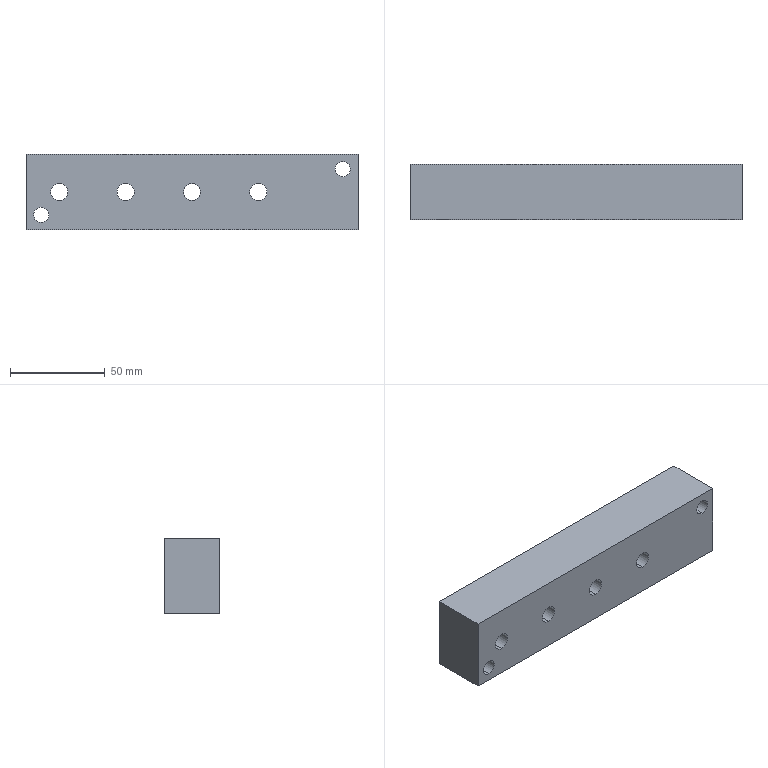Component | SolidWorks | Box151BackingPlateDiamondPin-1 | 1 solid | 33 faces | box 175 x 29 x 40 mm | volume 187063 mm3 | cylinder 22 | plane 11 | commonest cylinder face diameters 15 x8 9 x8 8 x4 10 x2
build123d program:
from build123d import *

# Parameters (mm, degrees)
SKETCH1_W                                       = 175
SKETCH1_H                                       = 40
BOSS_EXTRUDE1_DEPTH                             = 29
SKETCH2_R                                       = 5
CUT_EXTRUDE1_DEPTH                              = 20
M8_HEX_SOCKET_HEAD_CAP_SCREW_CBORE1_D           = 9
M8_HEX_SOCKET_HEAD_CAP_SCREW_CBORE1_CBORE_D     = 15
M8_HEX_SOCKET_HEAD_CAP_SCREW_CBORE1_CBORE_DEPTH = 9
SKETCH6_R                                       = 4
CUT_EXTRUDE2_DEPTH                              = 50


with BuildPart() as part:
    # Sketch1 → Boss-Extrude1 (new body)
    with BuildSketch(Plane(origin=(0, 0, 0), x_dir=(1, 0, 0), z_dir=(0, 1, 0))):
        Rectangle(SKETCH1_W, SKETCH1_H)
    extrude(amount=BOSS_EXTRUDE1_DEPTH)

    # Sketch2 → Cut-Extrude1 (cut)
    with BuildSketch(Plane(origin=(0, 29, 0), x_dir=(1, 0, 0), z_dir=(0, 1, 0))):
        with Locations(Location((-67, 2, 0), (0, 0, 270))):
            Circle(SKETCH2_R)
    extrude(amount=-CUT_EXTRUDE1_DEPTH, mode=Mode.SUBTRACT)

    # M8 Hex Socket Head Cap Screw CBORE1 (through all)
    with Locations(Plane(origin=(0, 29, 0), x_dir=(1, 0, 0), z_dir=(0, 1, 0))):
        with Locations((-35, 0), (0, 0), (35, 0), (70, 0)):
            CounterBoreHole(M8_HEX_SOCKET_HEAD_CAP_SCREW_CBORE1_D / 2, M8_HEX_SOCKET_HEAD_CAP_SCREW_CBORE1_CBORE_D / 2, M8_HEX_SOCKET_HEAD_CAP_SCREW_CBORE1_CBORE_DEPTH)

    # Sketch6 → Cut-Extrude2 (cut)
    with BuildSketch(Plane(origin=(0, 29, 0), x_dir=(1, 0, 0), z_dir=(0, 1, 0))):
        with Locations(Location((-79.5, 12, 0), (0, 0, 270))):
            Circle(SKETCH6_R)
        with Locations(Location((79.5, -12, 0), (0, 0, 270))):
            Circle(SKETCH6_R)
    extrude(amount=-CUT_EXTRUDE2_DEPTH, mode=Mode.SUBTRACT)


solid = part.part

# Placed as in the assembly
solid = solid.moved(Location((-3.619, 64.047, 50), (-180, 0, 180)))
STEP:
#1=CARTESIAN_POINT('',(2.987,2.522,2.283));
#2=VERTEX_POINT('',#1);
#3=CARTESIAN_POINT('',(2.987,2.522,2.598));
#4=VERTEX_POINT('',#3);
#5=CARTESIAN_POINT('',(2.987,2.522,2.441));
#6=DIRECTION('',(0.,-1.,0.));
#7=DIRECTION('',(0.,0.,1.));
#8=AXIS2_PLACEMENT_3D('',#5,#6,#7);
#9=CIRCLE('',#8,0.1575);
#10=EDGE_CURVE('',#2,#4,#9,.T.);
#11=ORIENTED_EDGE('',*,*,#10,.T.);
#12=CARTESIAN_POINT('',(2.987,3.663,2.598));
#13=VERTEX_POINT('',#12);
#14=CARTESIAN_POINT('',(2.987,1.695,2.598));
#15=DIRECTION('',(0.,1.,0.));
#16=VECTOR('',#15,39.37);
#17=LINE('',#14,#16);
#18=EDGE_CURVE('',#4,#13,#17,.T.);
#19=ORIENTED_EDGE('',*,*,#18,.T.);
#20=CARTESIAN_POINT('',(2.987,3.663,2.283));
#21=VERTEX_POINT('',#20);
#22=CARTESIAN_POINT('',(2.987,3.663,2.441));
#23=DIRECTION('',(0.,1.,0.));
#24=DIRECTION('',(0.,0.,-1.));
#25=AXIS2_PLACEMENT_3D('',#22,#23,#24);
#26=CIRCLE('',#25,0.1575);
#27=EDGE_CURVE('',#13,#21,#26,.T.);
#28=ORIENTED_EDGE('',*,*,#27,.T.);
#29=CARTESIAN_POINT('',(2.987,1.695,2.283));
#30=DIRECTION('',(0.,1.,0.));
#31=VECTOR('',#30,39.37);
#32=LINE('',#29,#31);
#33=EDGE_CURVE('',#2,#21,#32,.T.);
#34=ORIENTED_EDGE('',*,*,#33,.F.);
#35=EDGE_LOOP('',(#11,#19,#28,#34));
#36=FACE_OUTER_BOUND('',#35,.T.);
#37=CARTESIAN_POINT('',(2.987,1.695,2.441));
#38=DIRECTION('',(0.,1.,0.));
#39=DIRECTION('',(0.,0.,-1.));
#40=AXIS2_PLACEMENT_3D('',#37,#38,#39);
#41=CYLINDRICAL_SURFACE('',#40,0.1575);
#42=ADVANCED_FACE('',(#36),#41,.F.);
#43=CARTESIAN_POINT('',(-3.272,2.522,1.339));
#44=VERTEX_POINT('',#43);
#45=CARTESIAN_POINT('',(-3.272,2.522,1.654));
#46=VERTEX_POINT('',#45);
#47=CARTESIAN_POINT('',(-3.272,2.522,1.496));
#48=DIRECTION('',(0.,-1.,0.));
#49=DIRECTION('',(0.,0.,1.));
#50=AXIS2_PLACEMENT_3D('',#47,#48,#49);
#51=CIRCLE('',#50,0.1575);
#52=EDGE_CURVE('',#44,#46,#51,.T.);
#53=ORIENTED_EDGE('',*,*,#52,.T.);
#54=CARTESIAN_POINT('',(-3.272,3.663,1.654));
#55=VERTEX_POINT('',#54);
#56=CARTESIAN_POINT('',(-3.272,1.695,1.654));
#57=DIRECTION('',(0.,1.,0.));
#58=VECTOR('',#57,39.37);
#59=LINE('',#56,#58);
#60=EDGE_CURVE('',#46,#55,#59,.T.);
#61=ORIENTED_EDGE('',*,*,#60,.T.);
#62=CARTESIAN_POINT('',(-3.272,3.663,1.339));
#63=VERTEX_POINT('',#62);
#64=CARTESIAN_POINT('',(-3.272,3.663,1.496));
#65=DIRECTION('',(0.,1.,0.));
#66=DIRECTION('',(0.,0.,-1.));
#67=AXIS2_PLACEMENT_3D('',#64,#65,#66);
#68=CIRCLE('',#67,0.1575);
#69=EDGE_CURVE('',#55,#63,#68,.T.);
#70=ORIENTED_EDGE('',*,*,#69,.T.);
#71=CARTESIAN_POINT('',(-3.272,1.695,1.339));
#72=DIRECTION('',(0.,1.,0.));
#73=VECTOR('',#72,39.37);
#74=LINE('',#71,#73);
#75=EDGE_CURVE('',#44,#63,#74,.T.);
#76=ORIENTED_EDGE('',*,*,#75,.F.);
#77=EDGE_LOOP('',(#53,#61,#70,#76));
#78=FACE_OUTER_BOUND('',#77,.T.);
#79=CARTESIAN_POINT('',(-3.272,1.695,1.496));
#80=DIRECTION('',(0.,1.,0.));
#81=DIRECTION('',(0.,0.,-1.));
#82=AXIS2_PLACEMENT_3D('',#79,#80,#81);
#83=CYLINDRICAL_SURFACE('',#82,0.1575);
#84=ADVANCED_FACE('',(#78),#83,.F.);
#85=CARTESIAN_POINT('',(1.235,3.309,2.264));
#86=VERTEX_POINT('',#85);
#87=CARTESIAN_POINT('',(1.235,3.309,1.673));
#88=VERTEX_POINT('',#87);
#89=CARTESIAN_POINT('',(1.235,3.309,1.969));
#90=DIRECTION('',(0.,1.,0.));
#91=DIRECTION('',(0.,0.,-1.));
#92=AXIS2_PLACEMENT_3D('',#89,#90,#91);
#93=CIRCLE('',#92,0.2953);
#94=EDGE_CURVE('',#86,#88,#93,.T.);
#95=ORIENTED_EDGE('',*,*,#94,.F.);
#96=CARTESIAN_POINT('',(1.235,3.663,2.264));
#97=VERTEX_POINT('',#96);
#98=CARTESIAN_POINT('',(1.235,3.663,2.264));
#99=DIRECTION('',(0.,1.,0.));
#100=VECTOR('',#99,39.37);
#101=LINE('',#98,#100);
#102=EDGE_CURVE('',#86,#97,#101,.T.);
#103=ORIENTED_EDGE('',*,*,#102,.T.);
#104=CARTESIAN_POINT('',(1.235,3.663,1.673));
#105=VERTEX_POINT('',#104);
#106=CARTESIAN_POINT('',(1.235,3.663,1.969));
#107=DIRECTION('',(0.,1.,0.));
#108=DIRECTION('',(0.,0.,-1.));
#109=AXIS2_PLACEMENT_3D('',#106,#107,#108);
#110=CIRCLE('',#109,0.2953);
#111=EDGE_CURVE('',#97,#105,#110,.T.);
#112=ORIENTED_EDGE('',*,*,#111,.T.);
#113=CARTESIAN_POINT('',(1.235,3.663,1.673));
#114=DIRECTION('',(0.,1.,0.));
#115=VECTOR('',#114,39.37);
#116=LINE('',#113,#115);
#117=EDGE_CURVE('',#88,#105,#116,.T.);
#118=ORIENTED_EDGE('',*,*,#117,.F.);
#119=EDGE_LOOP('',(#95,#103,#112,#118));
#120=FACE_OUTER_BOUND('',#119,.T.);
#121=CARTESIAN_POINT('',(1.235,3.663,1.969));
#122=DIRECTION('',(0.,1.,0.));
#123=DIRECTION('',(0.,0.,-1.));
#124=AXIS2_PLACEMENT_3D('',#121,#122,#123);
#125=CYLINDRICAL_SURFACE('',#124,0.2953);
#126=ADVANCED_FACE('',(#120),#125,.F.);
#127=CARTESIAN_POINT('',(1.235,2.522,1.791));
#128=VERTEX_POINT('',#127);
#129=CARTESIAN_POINT('',(1.235,2.522,2.146));
#130=VERTEX_POINT('',#129);
#131=CARTESIAN_POINT('',(1.235,2.522,1.969));
#132=DIRECTION('',(0.,-1.,0.));
#133=DIRECTION('',(0.,0.,1.));
#134=AXIS2_PLACEMENT_3D('',#131,#132,#133);
#135=CIRCLE('',#134,0.1772);
#136=EDGE_CURVE('',#128,#130,#135,.T.);
#137=ORIENTED_EDGE('',*,*,#136,.T.);
#138=CARTESIAN_POINT('',(1.235,3.309,2.146));
#139=VERTEX_POINT('',#138);
#140=CARTESIAN_POINT('',(1.235,3.663,2.146));
#141=DIRECTION('',(0.,1.,0.));
#142=VECTOR('',#141,39.37);
#143=LINE('',#140,#142);
#144=EDGE_CURVE('',#130,#139,#143,.T.);
#145=ORIENTED_EDGE('',*,*,#144,.T.);
#146=CARTESIAN_POINT('',(1.235,3.309,1.791));
#147=VERTEX_POINT('',#146);
#148=CARTESIAN_POINT('',(1.235,3.309,1.969));
#149=DIRECTION('',(0.,1.,0.));
#150=DIRECTION('',(0.,0.,-1.));
#151=AXIS2_PLACEMENT_3D('',#148,#149,#150);
#152=CIRCLE('',#151,0.1772);
#153=EDGE_CURVE('',#139,#147,#152,.T.);
#154=ORIENTED_EDGE('',*,*,#153,.T.);
#155=CARTESIAN_POINT('',(1.235,3.663,1.791));
#156=DIRECTION('',(0.,1.,0.));
#157=VECTOR('',#156,39.37);
#158=LINE('',#155,#157);
#159=EDGE_CURVE('',#128,#147,#158,.T.);
#160=ORIENTED_EDGE('',*,*,#159,.F.);
#161=EDGE_LOOP('',(#137,#145,#154,#160));
#162=FACE_OUTER_BOUND('',#161,.T.);
#163=CARTESIAN_POINT('',(1.235,3.663,1.969));
#164=DIRECTION('',(0.,1.,0.));
#165=DIRECTION('',(0.,0.,-1.));
#166=AXIS2_PLACEMENT_3D('',#163,#164,#165);
#167=CYLINDRICAL_SURFACE('',#166,0.1772);
#168=ADVANCED_FACE('',(#162),#167,.F.);
#169=CARTESIAN_POINT('',(-0.1425,3.309,2.264));
#170=VERTEX_POINT('',#169);
#171=CARTESIAN_POINT('',(-0.1425,3.309,1.673));
#172=VERTEX_POINT('',#171);
#173=CARTESIAN_POINT('',(-0.1425,3.309,1.969));
#174=DIRECTION('',(0.,1.,0.));
#175=DIRECTION('',(-0.,0.,-1.));
#176=AXIS2_PLACEMENT_3D('',#173,#174,#175);
#177=CIRCLE('',#176,0.2953);
#178=EDGE_CURVE('',#170,#172,#177,.T.);
#179=ORIENTED_EDGE('',*,*,#178,.F.);
#180=CARTESIAN_POINT('',(-0.1425,3.663,2.264));
#181=VERTEX_POINT('',#180);
#182=CARTESIAN_POINT('',(-0.1425,3.663,2.264));
#183=DIRECTION('',(0.,1.,0.));
#184=VECTOR('',#183,39.37);
#185=LINE('',#182,#184);
#186=EDGE_CURVE('',#170,#181,#185,.T.);
#187=ORIENTED_EDGE('',*,*,#186,.T.);
#188=CARTESIAN_POINT('',(-0.1425,3.663,1.673));
#189=VERTEX_POINT('',#188);
#190=CARTESIAN_POINT('',(-0.1425,3.663,1.969));
#191=DIRECTION('',(0.,1.,0.));
#192=DIRECTION('',(-0.,0.,-1.));
#193=AXIS2_PLACEMENT_3D('',#190,#191,#192);
#194=CIRCLE('',#193,0.2953);
#195=EDGE_CURVE('',#181,#189,#194,.T.);
#196=ORIENTED_EDGE('',*,*,#195,.T.);
#197=CARTESIAN_POINT('',(-0.1425,3.663,1.673));
#198=DIRECTION('',(0.,1.,0.));
#199=VECTOR('',#198,39.37);
#200=LINE('',#197,#199);
#201=EDGE_CURVE('',#172,#189,#200,.T.);
#202=ORIENTED_EDGE('',*,*,#201,.F.);
#203=EDGE_LOOP('',(#179,#187,#196,#202));
#204=FACE_OUTER_BOUND('',#203,.T.);
#205=CARTESIAN_POINT('',(-0.1425,3.663,1.969));
#206=DIRECTION('',(0.,1.,0.));
#207=DIRECTION('',(-0.,0.,-1.));
#208=AXIS2_PLACEMENT_3D('',#205,#206,#207);
#209=CYLINDRICAL_SURFACE('',#208,0.2953);
#210=ADVANCED_FACE('',(#204),#209,.F.);
#211=CARTESIAN_POINT('',(-0.1425,2.522,1.791));
#212=VERTEX_POINT('',#211);
#213=CARTESIAN_POINT('',(-0.1425,2.522,2.146));
#214=VERTEX_POINT('',#213);
#215=CARTESIAN_POINT('',(-0.1425,2.522,1.969));
#216=DIRECTION('',(0.,-1.,0.));
#217=DIRECTION('',(0.,0.,1.));
#218=AXIS2_PLACEMENT_3D('',#215,#216,#217);
#219=CIRCLE('',#218,0.1772);
#220=EDGE_CURVE('',#212,#214,#219,.T.);
#221=ORIENTED_EDGE('',*,*,#220,.T.);
#222=CARTESIAN_POINT('',(-0.1425,3.309,2.146));
#223=VERTEX_POINT('',#222);
#224=CARTESIAN_POINT('',(-0.1425,3.663,2.146));
#225=DIRECTION('',(0.,1.,0.));
#226=VECTOR('',#225,39.37);
#227=LINE('',#224,#226);
#228=EDGE_CURVE('',#214,#223,#227,.T.);
#229=ORIENTED_EDGE('',*,*,#228,.T.);
#230=CARTESIAN_POINT('',(-0.1425,3.309,1.791));
#231=VERTEX_POINT('',#230);
#232=CARTESIAN_POINT('',(-0.1425,3.309,1.969));
#233=DIRECTION('',(0.,1.,0.));
#234=DIRECTION('',(-0.,0.,-1.));
#235=AXIS2_PLACEMENT_3D('',#232,#233,#234);
#236=CIRCLE('',#235,0.1772);
#237=EDGE_CURVE('',#223,#231,#236,.T.);
#238=ORIENTED_EDGE('',*,*,#237,.T.);
#239=CARTESIAN_POINT('',(-0.1425,3.663,1.791));
#240=DIRECTION('',(0.,1.,0.));
#241=VECTOR('',#240,39.37);
#242=LINE('',#239,#241);
#243=EDGE_CURVE('',#212,#231,#242,.T.);
#244=ORIENTED_EDGE('',*,*,#243,.F.);
#245=EDGE_LOOP('',(#221,#229,#238,#244));
#246=FACE_OUTER_BOUND('',#245,.T.);
#247=CARTESIAN_POINT('',(-0.1425,3.663,1.969));
#248=DIRECTION('',(0.,1.,0.));
#249=DIRECTION('',(-0.,0.,-1.));
#250=AXIS2_PLACEMENT_3D('',#247,#248,#249);
#251=CYLINDRICAL_SURFACE('',#250,0.1772);
#252=ADVANCED_FACE('',(#246),#251,.F.);
#253=CARTESIAN_POINT('',(-1.52,3.309,2.264));
#254=VERTEX_POINT('',#253);
#255=CARTESIAN_POINT('',(-1.52,3.309,1.673));
#256=VERTEX_POINT('',#255);
#257=CARTESIAN_POINT('',(-1.52,3.309,1.969));
#258=DIRECTION('',(0.,1.,0.));
#259=DIRECTION('',(0.,0.,-1.));
#260=AXIS2_PLACEMENT_3D('',#257,#258,#259);
#261=CIRCLE('',#260,0.2953);
#262=EDGE_CURVE('',#254,#256,#261,.T.);
#263=ORIENTED_EDGE('',*,*,#262,.F.);
#264=CARTESIAN_POINT('',(-1.52,3.663,2.264));
#265=VERTEX_POINT('',#264);
#266=CARTESIAN_POINT('',(-1.52,3.663,2.264));
#267=DIRECTION('',(0.,1.,0.));
#268=VECTOR('',#267,39.37);
#269=LINE('',#266,#268);
#270=EDGE_CURVE('',#254,#265,#269,.T.);
#271=ORIENTED_EDGE('',*,*,#270,.T.);
#272=CARTESIAN_POINT('',(-1.52,3.663,1.673));
#273=VERTEX_POINT('',#272);
#274=CARTESIAN_POINT('',(-1.52,3.663,1.969));
#275=DIRECTION('',(0.,1.,0.));
#276=DIRECTION('',(0.,0.,-1.));
#277=AXIS2_PLACEMENT_3D('',#274,#275,#276);
#278=CIRCLE('',#277,0.2953);
#279=EDGE_CURVE('',#265,#273,#278,.T.);
#280=ORIENTED_EDGE('',*,*,#279,.T.);
#281=CARTESIAN_POINT('',(-1.52,3.663,1.673));
#282=DIRECTION('',(0.,1.,0.));
#283=VECTOR('',#282,39.37);
#284=LINE('',#281,#283);
#285=EDGE_CURVE('',#256,#273,#284,.T.);
#286=ORIENTED_EDGE('',*,*,#285,.F.);
#287=EDGE_LOOP('',(#263,#271,#280,#286));
#288=FACE_OUTER_BOUND('',#287,.T.);
#289=CARTESIAN_POINT('',(-1.52,3.663,1.969));
#290=DIRECTION('',(0.,1.,0.));
#291=DIRECTION('',(0.,0.,-1.));
#292=AXIS2_PLACEMENT_3D('',#289,#290,#291);
#293=CYLINDRICAL_SURFACE('',#292,0.2953);
#294=ADVANCED_FACE('',(#288),#293,.F.);
#295=CARTESIAN_POINT('',(-1.52,2.522,1.791));
#296=VERTEX_POINT('',#295);
#297=CARTESIAN_POINT('',(-1.52,2.522,2.146));
#298=VERTEX_POINT('',#297);
#299=CARTESIAN_POINT('',(-1.52,2.522,1.969));
#300=DIRECTION('',(0.,-1.,0.));
#301=DIRECTION('',(0.,0.,1.));
#302=AXIS2_PLACEMENT_3D('',#299,#300,#301);
#303=CIRCLE('',#302,0.1772);
#304=EDGE_CURVE('',#296,#298,#303,.T.);
#305=ORIENTED_EDGE('',*,*,#304,.T.);
#306=CARTESIAN_POINT('',(-1.52,3.309,2.146));
#307=VERTEX_POINT('',#306);
#308=CARTESIAN_POINT('',(-1.52,3.663,2.146));
#309=DIRECTION('',(0.,1.,0.));
#310=VECTOR('',#309,39.37);
#311=LINE('',#308,#310);
#312=EDGE_CURVE('',#298,#307,#311,.T.);
#313=ORIENTED_EDGE('',*,*,#312,.T.);
#314=CARTESIAN_POINT('',(-1.52,3.309,1.791));
#315=VERTEX_POINT('',#314);
#316=CARTESIAN_POINT('',(-1.52,3.309,1.969));
#317=DIRECTION('',(0.,1.,0.));
#318=DIRECTION('',(0.,0.,-1.));
#319=AXIS2_PLACEMENT_3D('',#316,#317,#318);
#320=CIRCLE('',#319,0.1772);
#321=EDGE_CURVE('',#307,#315,#320,.T.);
#322=ORIENTED_EDGE('',*,*,#321,.T.);
#323=CARTESIAN_POINT('',(-1.52,3.663,1.791));
#324=DIRECTION('',(0.,1.,0.));
#325=VECTOR('',#324,39.37);
#326=LINE('',#323,#325);
#327=EDGE_CURVE('',#296,#315,#326,.T.);
#328=ORIENTED_EDGE('',*,*,#327,.F.);
#329=EDGE_LOOP('',(#305,#313,#322,#328));
#330=FACE_OUTER_BOUND('',#329,.T.);
#331=CARTESIAN_POINT('',(-1.52,3.663,1.969));
#332=DIRECTION('',(0.,1.,0.));
#333=DIRECTION('',(0.,0.,-1.));
#334=AXIS2_PLACEMENT_3D('',#331,#332,#333);
#335=CYLINDRICAL_SURFACE('',#334,0.1772);
#336=ADVANCED_FACE('',(#330),#335,.F.);
#337=CARTESIAN_POINT('',(-2.898,3.309,2.264));
#338=VERTEX_POINT('',#337);
#339=CARTESIAN_POINT('',(-2.898,3.309,1.673));
#340=VERTEX_POINT('',#339);
#341=CARTESIAN_POINT('',(-2.898,3.309,1.969));
#342=DIRECTION('',(0.,1.,0.));
#343=DIRECTION('',(0.,0.,-1.));
#344=AXIS2_PLACEMENT_3D('',#341,#342,#343);
#345=CIRCLE('',#344,0.2953);
#346=EDGE_CURVE('',#338,#340,#345,.T.);
#347=ORIENTED_EDGE('',*,*,#346,.F.);
#348=CARTESIAN_POINT('',(-2.898,3.663,2.264));
#349=VERTEX_POINT('',#348);
#350=CARTESIAN_POINT('',(-2.898,3.663,2.264));
#351=DIRECTION('',(0.,1.,0.));
#352=VECTOR('',#351,39.37);
#353=LINE('',#350,#352);
#354=EDGE_CURVE('',#338,#349,#353,.T.);
#355=ORIENTED_EDGE('',*,*,#354,.T.);
#356=CARTESIAN_POINT('',(-2.898,3.663,1.673));
#357=VERTEX_POINT('',#356);
#358=CARTESIAN_POINT('',(-2.898,3.663,1.969));
#359=DIRECTION('',(0.,1.,0.));
#360=DIRECTION('',(0.,0.,-1.));
#361=AXIS2_PLACEMENT_3D('',#358,#359,#360);
#362=CIRCLE('',#361,0.2953);
#363=EDGE_CURVE('',#349,#357,#362,.T.);
#364=ORIENTED_EDGE('',*,*,#363,.T.);
#365=CARTESIAN_POINT('',(-2.898,3.663,1.673));
#366=DIRECTION('',(0.,1.,0.));
#367=VECTOR('',#366,39.37);
#368=LINE('',#365,#367);
#369=EDGE_CURVE('',#340,#357,#368,.T.);
#370=ORIENTED_EDGE('',*,*,#369,.F.);
#371=EDGE_LOOP('',(#347,#355,#364,#370));
#372=FACE_OUTER_BOUND('',#371,.T.);
#373=CARTESIAN_POINT('',(-2.898,3.663,1.969));
#374=DIRECTION('',(0.,1.,0.));
#375=DIRECTION('',(0.,0.,-1.));
#376=AXIS2_PLACEMENT_3D('',#373,#374,#375);
#377=CYLINDRICAL_SURFACE('',#376,0.2953);
#378=ADVANCED_FACE('',(#372),#377,.F.);
#379=CARTESIAN_POINT('',(-2.898,2.522,1.791));
#380=VERTEX_POINT('',#379);
#381=CARTESIAN_POINT('',(-2.898,2.522,2.146));
#382=VERTEX_POINT('',#381);
#383=CARTESIAN_POINT('',(-2.898,2.522,1.969));
#384=DIRECTION('',(0.,-1.,0.));
#385=DIRECTION('',(0.,0.,1.));
#386=AXIS2_PLACEMENT_3D('',#383,#384,#385);
#387=CIRCLE('',#386,0.1772);
#388=EDGE_CURVE('',#380,#382,#387,.T.);
#389=ORIENTED_EDGE('',*,*,#388,.T.);
#390=CARTESIAN_POINT('',(-2.898,3.309,2.146));
#391=VERTEX_POINT('',#390);
#392=CARTESIAN_POINT('',(-2.898,3.663,2.146));
#393=DIRECTION('',(0.,1.,0.));
#394=VECTOR('',#393,39.37);
#395=LINE('',#392,#394);
#396=EDGE_CURVE('',#382,#391,#395,.T.);
#397=ORIENTED_EDGE('',*,*,#396,.T.);
#398=CARTESIAN_POINT('',(-2.898,3.309,1.791));
#399=VERTEX_POINT('',#398);
#400=CARTESIAN_POINT('',(-2.898,3.309,1.969));
#401=DIRECTION('',(0.,1.,0.));
#402=DIRECTION('',(0.,0.,-1.));
#403=AXIS2_PLACEMENT_3D('',#400,#401,#402);
#404=CIRCLE('',#403,0.1772);
#405=EDGE_CURVE('',#391,#399,#404,.T.);
#406=ORIENTED_EDGE('',*,*,#405,.T.);
#407=CARTESIAN_POINT('',(-2.898,3.663,1.791));
#408=DIRECTION('',(0.,1.,0.));
#409=VECTOR('',#408,39.37);
#410=LINE('',#407,#409);
#411=EDGE_CURVE('',#380,#399,#410,.T.);
#412=ORIENTED_EDGE('',*,*,#411,.F.);
#413=EDGE_LOOP('',(#389,#397,#406,#412));
#414=FACE_OUTER_BOUND('',#413,.T.);
#415=CARTESIAN_POINT('',(-2.898,3.663,1.969));
#416=DIRECTION('',(0.,1.,0.));
#417=DIRECTION('',(0.,0.,-1.));
#418=AXIS2_PLACEMENT_3D('',#415,#416,#417);
#419=CYLINDRICAL_SURFACE('',#418,0.1772);
#420=ADVANCED_FACE('',(#414),#419,.F.);
#421=CARTESIAN_POINT('',(2.495,2.876,2.244));
#422=VERTEX_POINT('',#421);
#423=CARTESIAN_POINT('',(2.495,2.876,1.85));
#424=VERTEX_POINT('',#423);
#425=CARTESIAN_POINT('',(2.495,2.876,2.047));
#426=DIRECTION('',(0.,1.,0.));
#427=DIRECTION('',(0.,0.,-1.));
#428=AXIS2_PLACEMENT_3D('',#425,#426,#427);
#429=CIRCLE('',#428,0.1969);
#430=EDGE_CURVE('',#422,#424,#429,.T.);
#431=ORIENTED_EDGE('',*,*,#430,.F.);
#432=CARTESIAN_POINT('',(2.495,3.663,2.244));
#433=VERTEX_POINT('',#432);
#434=CARTESIAN_POINT('',(2.495,2.876,2.244));
#435=DIRECTION('',(0.,1.,0.));
#436=VECTOR('',#435,39.37);
#437=LINE('',#434,#436);
#438=EDGE_CURVE('',#422,#433,#437,.T.);
#439=ORIENTED_EDGE('',*,*,#438,.T.);
#440=CARTESIAN_POINT('',(2.495,3.663,1.85));
#441=VERTEX_POINT('',#440);
#442=CARTESIAN_POINT('',(2.495,3.663,2.047));
#443=DIRECTION('',(0.,1.,0.));
#444=DIRECTION('',(0.,0.,-1.));
#445=AXIS2_PLACEMENT_3D('',#442,#443,#444);
#446=CIRCLE('',#445,0.1969);
#447=EDGE_CURVE('',#433,#441,#446,.T.);
#448=ORIENTED_EDGE('',*,*,#447,.T.);
#449=CARTESIAN_POINT('',(2.495,2.876,1.85));
#450=DIRECTION('',(0.,1.,0.));
#451=VECTOR('',#450,39.37);
#452=LINE('',#449,#451);
#453=EDGE_CURVE('',#424,#441,#452,.T.);
#454=ORIENTED_EDGE('',*,*,#453,.F.);
#455=EDGE_LOOP('',(#431,#439,#448,#454));
#456=FACE_OUTER_BOUND('',#455,.T.);
#457=CARTESIAN_POINT('',(2.495,2.876,2.047));
#458=DIRECTION('',(0.,1.,0.));
#459=DIRECTION('',(0.,0.,-1.));
#460=AXIS2_PLACEMENT_3D('',#457,#458,#459);
#461=CYLINDRICAL_SURFACE('',#460,0.1969);
#462=ADVANCED_FACE('',(#456),#461,.F.);
#463=CARTESIAN_POINT('',(2.987,3.663,2.441));
#464=DIRECTION('',(0.,1.,0.));
#465=DIRECTION('',(0.,0.,-1.));
#466=AXIS2_PLACEMENT_3D('',#463,#464,#465);
#467=CIRCLE('',#466,0.1575);
#468=EDGE_CURVE('',#21,#13,#467,.T.);
#469=ORIENTED_EDGE('',*,*,#468,.F.);
#470=ORIENTED_EDGE('',*,*,#27,.F.);
#471=EDGE_LOOP('',(#469,#470));
#472=FACE_BOUND('',#471,.T.);
#473=CARTESIAN_POINT('',(-3.272,3.663,1.496));
#474=DIRECTION('',(0.,1.,0.));
#475=DIRECTION('',(0.,0.,-1.));
#476=AXIS2_PLACEMENT_3D('',#473,#474,#475);
#477=CIRCLE('',#476,0.1575);
#478=EDGE_CURVE('',#63,#55,#477,.T.);
#479=ORIENTED_EDGE('',*,*,#478,.F.);
#480=ORIENTED_EDGE('',*,*,#69,.F.);
#481=EDGE_LOOP('',(#479,#480));
#482=FACE_BOUND('',#481,.T.);
#483=CARTESIAN_POINT('',(-0.1425,3.663,1.969));
#484=DIRECTION('',(0.,1.,0.));
#485=DIRECTION('',(-0.,0.,-1.));
#486=AXIS2_PLACEMENT_3D('',#483,#484,#485);
#487=CIRCLE('',#486,0.2953);
#488=EDGE_CURVE('',#189,#181,#487,.T.);
#489=ORIENTED_EDGE('',*,*,#488,.F.);
#490=ORIENTED_EDGE('',*,*,#195,.F.);
#491=EDGE_LOOP('',(#489,#490));
#492=FACE_BOUND('',#491,.T.);
#493=CARTESIAN_POINT('',(-1.52,3.663,1.969));
#494=DIRECTION('',(0.,1.,0.));
#495=DIRECTION('',(0.,0.,-1.));
#496=AXIS2_PLACEMENT_3D('',#493,#494,#495);
#497=CIRCLE('',#496,0.2953);
#498=EDGE_CURVE('',#273,#265,#497,.T.);
#499=ORIENTED_EDGE('',*,*,#498,.F.);
#500=ORIENTED_EDGE('',*,*,#279,.F.);
#501=EDGE_LOOP('',(#499,#500));
#502=FACE_BOUND('',#501,.T.);
#503=CARTESIAN_POINT('',(-2.898,3.663,1.969));
#504=DIRECTION('',(0.,1.,0.));
#505=DIRECTION('',(0.,0.,-1.));
#506=AXIS2_PLACEMENT_3D('',#503,#504,#505);
#507=CIRCLE('',#506,0.2953);
#508=EDGE_CURVE('',#357,#349,#507,.T.);
#509=ORIENTED_EDGE('',*,*,#508,.F.);
#510=ORIENTED_EDGE('',*,*,#363,.F.);
#511=EDGE_LOOP('',(#509,#510));
#512=FACE_BOUND('',#511,.T.);
#513=CARTESIAN_POINT('',(2.495,3.663,2.047));
#514=DIRECTION('',(0.,1.,0.));
#515=DIRECTION('',(0.,0.,-1.));
#516=AXIS2_PLACEMENT_3D('',#513,#514,#515);
#517=CIRCLE('',#516,0.1969);
#518=EDGE_CURVE('',#441,#433,#517,.T.);
#519=ORIENTED_EDGE('',*,*,#518,.F.);
#520=ORIENTED_EDGE('',*,*,#447,.F.);
#521=EDGE_LOOP('',(#519,#520));
#522=FACE_BOUND('',#521,.T.);
#523=CARTESIAN_POINT('',(-3.587,3.663,1.181));
#524=VERTEX_POINT('',#523);
#525=CARTESIAN_POINT('',(-3.587,3.663,2.756));
#526=VERTEX_POINT('',#525);
#527=CARTESIAN_POINT('',(-3.587,3.663,1.181));
#528=DIRECTION('',(0.,0.,1.));
#529=VECTOR('',#528,39.37);
#530=LINE('',#527,#529);
#531=EDGE_CURVE('',#524,#526,#530,.T.);
#532=ORIENTED_EDGE('',*,*,#531,.T.);
#533=CARTESIAN_POINT('',(3.302,3.663,2.756));
#534=VERTEX_POINT('',#533);
#535=CARTESIAN_POINT('',(3.302,3.663,2.756));
#536=DIRECTION('',(1.,0.,-0.));
#537=VECTOR('',#536,39.37);
#538=LINE('',#535,#537);
#539=EDGE_CURVE('',#526,#534,#538,.T.);
#540=ORIENTED_EDGE('',*,*,#539,.T.);
#541=CARTESIAN_POINT('',(3.302,3.663,1.181));
#542=VERTEX_POINT('',#541);
#543=CARTESIAN_POINT('',(3.302,3.663,1.181));
#544=DIRECTION('',(-0.,0.,-1.));
#545=VECTOR('',#544,39.37);
#546=LINE('',#543,#545);
#547=EDGE_CURVE('',#534,#542,#546,.T.);
#548=ORIENTED_EDGE('',*,*,#547,.T.);
#549=CARTESIAN_POINT('',(3.302,3.663,1.181));
#550=DIRECTION('',(-1.,0.,0.));
#551=VECTOR('',#550,39.37);
#552=LINE('',#549,#551);
#553=EDGE_CURVE('',#542,#524,#552,.T.);
#554=ORIENTED_EDGE('',*,*,#553,.T.);
#555=EDGE_LOOP('',(#532,#540,#548,#554));
#556=FACE_OUTER_BOUND('',#555,.T.);
#557=CARTESIAN_POINT('',(1.235,3.663,1.969));
#558=DIRECTION('',(0.,1.,0.));
#559=DIRECTION('',(0.,0.,-1.));
#560=AXIS2_PLACEMENT_3D('',#557,#558,#559);
#561=CIRCLE('',#560,0.2953);
#562=EDGE_CURVE('',#105,#97,#561,.T.);
#563=ORIENTED_EDGE('',*,*,#562,.F.);
#564=ORIENTED_EDGE('',*,*,#111,.F.);
#565=EDGE_LOOP('',(#563,#564));
#566=FACE_BOUND('',#565,.T.);
#567=CARTESIAN_POINT('',(-0.1425,3.663,1.969));
#568=DIRECTION('',(0.,-1.,0.));
#569=DIRECTION('',(0.,0.,1.));
#570=AXIS2_PLACEMENT_3D('',#567,#568,#569);
#571=PLANE('',#570);
#572=ADVANCED_FACE('',(#472,#482,#492,#502,#512,#522,#556,#566),#571,.F.);
#573=CARTESIAN_POINT('',(-3.587,2.522,1.181));
#574=VERTEX_POINT('',#573);
#575=CARTESIAN_POINT('',(-3.587,2.522,2.756));
#576=VERTEX_POINT('',#575);
#577=CARTESIAN_POINT('',(-3.587,2.522,1.181));
#578=DIRECTION('',(0.,0.,1.));
#579=VECTOR('',#578,39.37);
#580=LINE('',#577,#579);
#581=EDGE_CURVE('',#574,#576,#580,.T.);
#582=ORIENTED_EDGE('',*,*,#581,.T.);
#583=CARTESIAN_POINT('',(-3.587,3.663,2.756));
#584=DIRECTION('',(0.,-1.,0.));
#585=VECTOR('',#584,39.37);
#586=LINE('',#583,#585);
#587=EDGE_CURVE('',#526,#576,#586,.T.);
#588=ORIENTED_EDGE('',*,*,#587,.F.);
#589=ORIENTED_EDGE('',*,*,#531,.F.);
#590=CARTESIAN_POINT('',(-3.587,3.663,1.181));
#591=DIRECTION('',(0.,-1.,0.));
#592=VECTOR('',#591,39.37);
#593=LINE('',#590,#592);
#594=EDGE_CURVE('',#524,#574,#593,.T.);
#595=ORIENTED_EDGE('',*,*,#594,.T.);
#596=EDGE_LOOP('',(#582,#588,#589,#595));
#597=FACE_OUTER_BOUND('',#596,.T.);
#598=CARTESIAN_POINT('',(-3.587,3.663,1.181));
#599=DIRECTION('',(1.,0.,-0.));
#600=DIRECTION('',(-0.,0.,-1.));
#601=AXIS2_PLACEMENT_3D('',#598,#599,#600);
#602=PLANE('',#601);
#603=ADVANCED_FACE('',(#597),#602,.F.);
#604=CARTESIAN_POINT('',(3.302,2.522,2.756));
#605=VERTEX_POINT('',#604);
#606=CARTESIAN_POINT('',(3.302,2.522,2.756));
#607=DIRECTION('',(1.,0.,-0.));
#608=VECTOR('',#607,39.37);
#609=LINE('',#606,#608);
#610=EDGE_CURVE('',#576,#605,#609,.T.);
#611=ORIENTED_EDGE('',*,*,#610,.T.);
#612=CARTESIAN_POINT('',(3.302,3.663,2.756));
#613=DIRECTION('',(0.,-1.,0.));
#614=VECTOR('',#613,39.37);
#615=LINE('',#612,#614);
#616=EDGE_CURVE('',#534,#605,#615,.T.);
#617=ORIENTED_EDGE('',*,*,#616,.F.);
#618=ORIENTED_EDGE('',*,*,#539,.F.);
#619=ORIENTED_EDGE('',*,*,#587,.T.);
#620=EDGE_LOOP('',(#611,#617,#618,#619));
#621=FACE_OUTER_BOUND('',#620,.T.);
#622=CARTESIAN_POINT('',(3.302,3.663,2.756));
#623=DIRECTION('',(-0.,0.,-1.));
#624=DIRECTION('',(-1.,0.,0.));
#625=AXIS2_PLACEMENT_3D('',#622,#623,#624);
#626=PLANE('',#625);
#627=ADVANCED_FACE('',(#621),#626,.F.);
#628=CARTESIAN_POINT('',(3.302,2.522,1.181));
#629=VERTEX_POINT('',#628);
#630=CARTESIAN_POINT('',(3.302,2.522,1.181));
#631=DIRECTION('',(-0.,0.,-1.));
#632=VECTOR('',#631,39.37);
#633=LINE('',#630,#632);
#634=EDGE_CURVE('',#605,#629,#633,.T.);
#635=ORIENTED_EDGE('',*,*,#634,.T.);
#636=CARTESIAN_POINT('',(3.302,3.663,1.181));
#637=DIRECTION('',(0.,-1.,0.));
#638=VECTOR('',#637,39.37);
#639=LINE('',#636,#638);
#640=EDGE_CURVE('',#542,#629,#639,.T.);
#641=ORIENTED_EDGE('',*,*,#640,.F.);
#642=ORIENTED_EDGE('',*,*,#547,.F.);
#643=ORIENTED_EDGE('',*,*,#616,.T.);
#644=EDGE_LOOP('',(#635,#641,#642,#643));
#645=FACE_OUTER_BOUND('',#644,.T.);
#646=CARTESIAN_POINT('',(3.302,3.663,1.181));
#647=DIRECTION('',(-1.,0.,0.));
#648=DIRECTION('',(0.,0.,1.));
#649=AXIS2_PLACEMENT_3D('',#646,#647,#648);
#650=PLANE('',#649);
#651=ADVANCED_FACE('',(#645),#650,.F.);
#652=CARTESIAN_POINT('',(3.302,2.522,1.181));
#653=DIRECTION('',(-1.,0.,0.));
#654=VECTOR('',#653,39.37);
#655=LINE('',#652,#654);
#656=EDGE_CURVE('',#629,#574,#655,.T.);
#657=ORIENTED_EDGE('',*,*,#656,.T.);
#658=ORIENTED_EDGE('',*,*,#594,.F.);
#659=ORIENTED_EDGE('',*,*,#553,.F.);
#660=ORIENTED_EDGE('',*,*,#640,.T.);
#661=EDGE_LOOP('',(#657,#658,#659,#660));
#662=FACE_OUTER_BOUND('',#661,.T.);
#663=CARTESIAN_POINT('',(3.302,3.663,1.181));
#664=DIRECTION('',(0.,0.,1.));
#665=DIRECTION('',(1.,0.,-0.));
#666=AXIS2_PLACEMENT_3D('',#663,#664,#665);
#667=PLANE('',#666);
#668=ADVANCED_FACE('',(#662),#667,.F.);
#669=ORIENTED_EDGE('',*,*,#10,.F.);
#670=CARTESIAN_POINT('',(2.987,2.522,2.441));
#671=DIRECTION('',(0.,-1.,0.));
#672=DIRECTION('',(0.,0.,1.));
#673=AXIS2_PLACEMENT_3D('',#670,#671,#672);
#674=CIRCLE('',#673,0.1575);
#675=EDGE_CURVE('',#4,#2,#674,.T.);
#676=ORIENTED_EDGE('',*,*,#675,.F.);
#677=EDGE_LOOP('',(#669,#676));
#678=FACE_BOUND('',#677,.T.);
#679=ORIENTED_EDGE('',*,*,#52,.F.);
#680=CARTESIAN_POINT('',(-3.272,2.522,1.496));
#681=DIRECTION('',(0.,-1.,0.));
#682=DIRECTION('',(0.,0.,1.));
#683=AXIS2_PLACEMENT_3D('',#680,#681,#682);
#684=CIRCLE('',#683,0.1575);
#685=EDGE_CURVE('',#46,#44,#684,.T.);
#686=ORIENTED_EDGE('',*,*,#685,.F.);
#687=EDGE_LOOP('',(#679,#686));
#688=FACE_BOUND('',#687,.T.);
#689=ORIENTED_EDGE('',*,*,#136,.F.);
#690=CARTESIAN_POINT('',(1.235,2.522,1.969));
#691=DIRECTION('',(0.,-1.,0.));
#692=DIRECTION('',(0.,0.,1.));
#693=AXIS2_PLACEMENT_3D('',#690,#691,#692);
#694=CIRCLE('',#693,0.1772);
#695=EDGE_CURVE('',#130,#128,#694,.T.);
#696=ORIENTED_EDGE('',*,*,#695,.F.);
#697=EDGE_LOOP('',(#689,#696));
#698=FACE_BOUND('',#697,.T.);
#699=ORIENTED_EDGE('',*,*,#220,.F.);
#700=CARTESIAN_POINT('',(-0.1425,2.522,1.969));
#701=DIRECTION('',(0.,-1.,0.));
#702=DIRECTION('',(0.,0.,1.));
#703=AXIS2_PLACEMENT_3D('',#700,#701,#702);
#704=CIRCLE('',#703,0.1772);
#705=EDGE_CURVE('',#214,#212,#704,.T.);
#706=ORIENTED_EDGE('',*,*,#705,.F.);
#707=EDGE_LOOP('',(#699,#706));
#708=FACE_BOUND('',#707,.T.);
#709=ORIENTED_EDGE('',*,*,#304,.F.);
#710=CARTESIAN_POINT('',(-1.52,2.522,1.969));
#711=DIRECTION('',(0.,-1.,0.));
#712=DIRECTION('',(0.,0.,1.));
#713=AXIS2_PLACEMENT_3D('',#710,#711,#712);
#714=CIRCLE('',#713,0.1772);
#715=EDGE_CURVE('',#298,#296,#714,.T.);
#716=ORIENTED_EDGE('',*,*,#715,.F.);
#717=EDGE_LOOP('',(#709,#716));
#718=FACE_BOUND('',#717,.T.);
#719=ORIENTED_EDGE('',*,*,#388,.F.);
#720=CARTESIAN_POINT('',(-2.898,2.522,1.969));
#721=DIRECTION('',(0.,-1.,0.));
#722=DIRECTION('',(0.,0.,1.));
#723=AXIS2_PLACEMENT_3D('',#720,#721,#722);
#724=CIRCLE('',#723,0.1772);
#725=EDGE_CURVE('',#382,#380,#724,.T.);
#726=ORIENTED_EDGE('',*,*,#725,.F.);
#727=EDGE_LOOP('',(#719,#726));
#728=FACE_BOUND('',#727,.T.);
#729=ORIENTED_EDGE('',*,*,#581,.F.);
#730=ORIENTED_EDGE('',*,*,#656,.F.);
#731=ORIENTED_EDGE('',*,*,#634,.F.);
#732=ORIENTED_EDGE('',*,*,#610,.F.);
#733=EDGE_LOOP('',(#729,#730,#731,#732));
#734=FACE_OUTER_BOUND('',#733,.T.);
#735=CARTESIAN_POINT('',(-0.1425,2.522,1.969));
#736=DIRECTION('',(0.,-1.,0.));
#737=DIRECTION('',(0.,0.,1.));
#738=AXIS2_PLACEMENT_3D('',#735,#736,#737);
#739=PLANE('',#738);
#740=ADVANCED_FACE('',(#678,#688,#698,#708,#718,#728,#734),#739,.T.);
#741=ORIENTED_EDGE('',*,*,#438,.F.);
#742=CARTESIAN_POINT('',(2.495,2.876,2.047));
#743=DIRECTION('',(0.,1.,0.));
#744=DIRECTION('',(0.,0.,-1.));
#745=AXIS2_PLACEMENT_3D('',#742,#743,#744);
#746=CIRCLE('',#745,0.1969);
#747=EDGE_CURVE('',#424,#422,#746,.T.);
#748=ORIENTED_EDGE('',*,*,#747,.F.);
#749=ORIENTED_EDGE('',*,*,#453,.T.);
#750=ORIENTED_EDGE('',*,*,#518,.T.);
#751=EDGE_LOOP('',(#741,#748,#749,#750));
#752=FACE_OUTER_BOUND('',#751,.T.);
#753=CARTESIAN_POINT('',(2.495,2.876,2.047));
#754=DIRECTION('',(0.,1.,0.));
#755=DIRECTION('',(0.,0.,-1.));
#756=AXIS2_PLACEMENT_3D('',#753,#754,#755);
#757=CYLINDRICAL_SURFACE('',#756,0.1969);
#758=ADVANCED_FACE('',(#752),#757,.F.);
#759=ORIENTED_EDGE('',*,*,#747,.T.);
#760=ORIENTED_EDGE('',*,*,#430,.T.);
#761=EDGE_LOOP('',(#759,#760));
#762=FACE_OUTER_BOUND('',#761,.T.);
#763=CARTESIAN_POINT('',(2.495,2.876,2.047));
#764=DIRECTION('',(0.,1.,0.));
#765=DIRECTION('',(-0.,0.,-1.));
#766=AXIS2_PLACEMENT_3D('',#763,#764,#765);
#767=PLANE('',#766);
#768=ADVANCED_FACE('',(#762),#767,.T.);
#769=ORIENTED_EDGE('',*,*,#396,.F.);
#770=ORIENTED_EDGE('',*,*,#725,.T.);
#771=ORIENTED_EDGE('',*,*,#411,.T.);
#772=CARTESIAN_POINT('',(-2.898,3.309,1.969));
#773=DIRECTION('',(0.,1.,0.));
#774=DIRECTION('',(0.,0.,-1.));
#775=AXIS2_PLACEMENT_3D('',#772,#773,#774);
#776=CIRCLE('',#775,0.1772);
#777=EDGE_CURVE('',#399,#391,#776,.T.);
#778=ORIENTED_EDGE('',*,*,#777,.T.);
#779=EDGE_LOOP('',(#769,#770,#771,#778));
#780=FACE_OUTER_BOUND('',#779,.T.);
#781=CARTESIAN_POINT('',(-2.898,3.663,1.969));
#782=DIRECTION('',(0.,1.,0.));
#783=DIRECTION('',(0.,0.,-1.));
#784=AXIS2_PLACEMENT_3D('',#781,#782,#783);
#785=CYLINDRICAL_SURFACE('',#784,0.1772);
#786=ADVANCED_FACE('',(#780),#785,.F.);
#787=ORIENTED_EDGE('',*,*,#777,.F.);
#788=ORIENTED_EDGE('',*,*,#405,.F.);
#789=EDGE_LOOP('',(#787,#788));
#790=FACE_BOUND('',#789,.T.);
#791=CARTESIAN_POINT('',(-2.898,3.309,1.969));
#792=DIRECTION('',(0.,1.,0.));
#793=DIRECTION('',(0.,0.,-1.));
#794=AXIS2_PLACEMENT_3D('',#791,#792,#793);
#795=CIRCLE('',#794,0.2953);
#796=EDGE_CURVE('',#340,#338,#795,.T.);
#797=ORIENTED_EDGE('',*,*,#796,.T.);
#798=ORIENTED_EDGE('',*,*,#346,.T.);
#799=EDGE_LOOP('',(#797,#798));
#800=FACE_OUTER_BOUND('',#799,.T.);
#801=CARTESIAN_POINT('',(-3.076,3.309,1.969));
#802=DIRECTION('',(0.,-1.,0.));
#803=DIRECTION('',(0.,0.,1.));
#804=AXIS2_PLACEMENT_3D('',#801,#802,#803);
#805=PLANE('',#804);
#806=ADVANCED_FACE('',(#790,#800),#805,.F.);
#807=ORIENTED_EDGE('',*,*,#354,.F.);
#808=ORIENTED_EDGE('',*,*,#796,.F.);
#809=ORIENTED_EDGE('',*,*,#369,.T.);
#810=ORIENTED_EDGE('',*,*,#508,.T.);
#811=EDGE_LOOP('',(#807,#808,#809,#810));
#812=FACE_OUTER_BOUND('',#811,.T.);
#813=CARTESIAN_POINT('',(-2.898,3.663,1.969));
#814=DIRECTION('',(0.,1.,0.));
#815=DIRECTION('',(0.,0.,-1.));
#816=AXIS2_PLACEMENT_3D('',#813,#814,#815);
#817=CYLINDRICAL_SURFACE('',#816,0.2953);
#818=ADVANCED_FACE('',(#812),#817,.F.);
#819=ORIENTED_EDGE('',*,*,#312,.F.);
#820=ORIENTED_EDGE('',*,*,#715,.T.);
#821=ORIENTED_EDGE('',*,*,#327,.T.);
#822=CARTESIAN_POINT('',(-1.52,3.309,1.969));
#823=DIRECTION('',(0.,1.,0.));
#824=DIRECTION('',(0.,0.,-1.));
#825=AXIS2_PLACEMENT_3D('',#822,#823,#824);
#826=CIRCLE('',#825,0.1772);
#827=EDGE_CURVE('',#315,#307,#826,.T.);
#828=ORIENTED_EDGE('',*,*,#827,.T.);
#829=EDGE_LOOP('',(#819,#820,#821,#828));
#830=FACE_OUTER_BOUND('',#829,.T.);
#831=CARTESIAN_POINT('',(-1.52,3.663,1.969));
#832=DIRECTION('',(0.,1.,0.));
#833=DIRECTION('',(0.,0.,-1.));
#834=AXIS2_PLACEMENT_3D('',#831,#832,#833);
#835=CYLINDRICAL_SURFACE('',#834,0.1772);
#836=ADVANCED_FACE('',(#830),#835,.F.);
#837=ORIENTED_EDGE('',*,*,#827,.F.);
#838=ORIENTED_EDGE('',*,*,#321,.F.);
#839=EDGE_LOOP('',(#837,#838));
#840=FACE_BOUND('',#839,.T.);
#841=CARTESIAN_POINT('',(-1.52,3.309,1.969));
#842=DIRECTION('',(0.,1.,0.));
#843=DIRECTION('',(0.,0.,-1.));
#844=AXIS2_PLACEMENT_3D('',#841,#842,#843);
#845=CIRCLE('',#844,0.2953);
#846=EDGE_CURVE('',#256,#254,#845,.T.);
#847=ORIENTED_EDGE('',*,*,#846,.T.);
#848=ORIENTED_EDGE('',*,*,#262,.T.);
#849=EDGE_LOOP('',(#847,#848));
#850=FACE_OUTER_BOUND('',#849,.T.);
#851=CARTESIAN_POINT('',(-1.698,3.309,1.969));
#852=DIRECTION('',(0.,-1.,0.));
#853=DIRECTION('',(0.,0.,1.));
#854=AXIS2_PLACEMENT_3D('',#851,#852,#853);
#855=PLANE('',#854);
#856=ADVANCED_FACE('',(#840,#850),#855,.F.);
#857=ORIENTED_EDGE('',*,*,#270,.F.);
#858=ORIENTED_EDGE('',*,*,#846,.F.);
#859=ORIENTED_EDGE('',*,*,#285,.T.);
#860=ORIENTED_EDGE('',*,*,#498,.T.);
#861=EDGE_LOOP('',(#857,#858,#859,#860));
#862=FACE_OUTER_BOUND('',#861,.T.);
#863=CARTESIAN_POINT('',(-1.52,3.663,1.969));
#864=DIRECTION('',(0.,1.,0.));
#865=DIRECTION('',(0.,0.,-1.));
#866=AXIS2_PLACEMENT_3D('',#863,#864,#865);
#867=CYLINDRICAL_SURFACE('',#866,0.2953);
#868=ADVANCED_FACE('',(#862),#867,.F.);
#869=ORIENTED_EDGE('',*,*,#228,.F.);
#870=ORIENTED_EDGE('',*,*,#705,.T.);
#871=ORIENTED_EDGE('',*,*,#243,.T.);
#872=CARTESIAN_POINT('',(-0.1425,3.309,1.969));
#873=DIRECTION('',(0.,1.,0.));
#874=DIRECTION('',(-0.,0.,-1.));
#875=AXIS2_PLACEMENT_3D('',#872,#873,#874);
#876=CIRCLE('',#875,0.1772);
#877=EDGE_CURVE('',#231,#223,#876,.T.);
#878=ORIENTED_EDGE('',*,*,#877,.T.);
#879=EDGE_LOOP('',(#869,#870,#871,#878));
#880=FACE_OUTER_BOUND('',#879,.T.);
#881=CARTESIAN_POINT('',(-0.1425,3.663,1.969));
#882=DIRECTION('',(0.,1.,0.));
#883=DIRECTION('',(-0.,0.,-1.));
#884=AXIS2_PLACEMENT_3D('',#881,#882,#883);
#885=CYLINDRICAL_SURFACE('',#884,0.1772);
#886=ADVANCED_FACE('',(#880),#885,.F.);
#887=ORIENTED_EDGE('',*,*,#877,.F.);
#888=ORIENTED_EDGE('',*,*,#237,.F.);
#889=EDGE_LOOP('',(#887,#888));
#890=FACE_BOUND('',#889,.T.);
#891=CARTESIAN_POINT('',(-0.1425,3.309,1.969));
#892=DIRECTION('',(0.,1.,0.));
#893=DIRECTION('',(-0.,0.,-1.));
#894=AXIS2_PLACEMENT_3D('',#891,#892,#893);
#895=CIRCLE('',#894,0.2953);
#896=EDGE_CURVE('',#172,#170,#895,.T.);
#897=ORIENTED_EDGE('',*,*,#896,.T.);
#898=ORIENTED_EDGE('',*,*,#178,.T.);
#899=EDGE_LOOP('',(#897,#898));
#900=FACE_OUTER_BOUND('',#899,.T.);
#901=CARTESIAN_POINT('',(-0.3196,3.309,1.969));
#902=DIRECTION('',(0.,-1.,0.));
#903=DIRECTION('',(0.,0.,1.));
#904=AXIS2_PLACEMENT_3D('',#901,#902,#903);
#905=PLANE('',#904);
#906=ADVANCED_FACE('',(#890,#900),#905,.F.);
#907=ORIENTED_EDGE('',*,*,#186,.F.);
#908=ORIENTED_EDGE('',*,*,#896,.F.);
#909=ORIENTED_EDGE('',*,*,#201,.T.);
#910=ORIENTED_EDGE('',*,*,#488,.T.);
#911=EDGE_LOOP('',(#907,#908,#909,#910));
#912=FACE_OUTER_BOUND('',#911,.T.);
#913=CARTESIAN_POINT('',(-0.1425,3.663,1.969));
#914=DIRECTION('',(0.,1.,0.));
#915=DIRECTION('',(-0.,0.,-1.));
#916=AXIS2_PLACEMENT_3D('',#913,#914,#915);
#917=CYLINDRICAL_SURFACE('',#916,0.2953);
#918=ADVANCED_FACE('',(#912),#917,.F.);
#919=ORIENTED_EDGE('',*,*,#144,.F.);
#920=ORIENTED_EDGE('',*,*,#695,.T.);
#921=ORIENTED_EDGE('',*,*,#159,.T.);
#922=CARTESIAN_POINT('',(1.235,3.309,1.969));
#923=DIRECTION('',(0.,1.,0.));
#924=DIRECTION('',(0.,0.,-1.));
#925=AXIS2_PLACEMENT_3D('',#922,#923,#924);
#926=CIRCLE('',#925,0.1772);
#927=EDGE_CURVE('',#147,#139,#926,.T.);
#928=ORIENTED_EDGE('',*,*,#927,.T.);
#929=EDGE_LOOP('',(#919,#920,#921,#928));
#930=FACE_OUTER_BOUND('',#929,.T.);
#931=CARTESIAN_POINT('',(1.235,3.663,1.969));
#932=DIRECTION('',(0.,1.,0.));
#933=DIRECTION('',(0.,0.,-1.));
#934=AXIS2_PLACEMENT_3D('',#931,#932,#933);
#935=CYLINDRICAL_SURFACE('',#934,0.1772);
#936=ADVANCED_FACE('',(#930),#935,.F.);
#937=ORIENTED_EDGE('',*,*,#927,.F.);
#938=ORIENTED_EDGE('',*,*,#153,.F.);
#939=EDGE_LOOP('',(#937,#938));
#940=FACE_BOUND('',#939,.T.);
#941=CARTESIAN_POINT('',(1.235,3.309,1.969));
#942=DIRECTION('',(0.,1.,0.));
#943=DIRECTION('',(0.,0.,-1.));
#944=AXIS2_PLACEMENT_3D('',#941,#942,#943);
#945=CIRCLE('',#944,0.2953);
#946=EDGE_CURVE('',#88,#86,#945,.T.);
#947=ORIENTED_EDGE('',*,*,#946,.T.);
#948=ORIENTED_EDGE('',*,*,#94,.T.);
#949=EDGE_LOOP('',(#947,#948));
#950=FACE_OUTER_BOUND('',#949,.T.);
#951=CARTESIAN_POINT('',(1.058,3.309,1.969));
#952=DIRECTION('',(0.,-1.,0.));
#953=DIRECTION('',(0.,0.,1.));
#954=AXIS2_PLACEMENT_3D('',#951,#952,#953);
#955=PLANE('',#954);
#956=ADVANCED_FACE('',(#940,#950),#955,.F.);
#957=ORIENTED_EDGE('',*,*,#102,.F.);
#958=ORIENTED_EDGE('',*,*,#946,.F.);
#959=ORIENTED_EDGE('',*,*,#117,.T.);
#960=ORIENTED_EDGE('',*,*,#562,.T.);
#961=EDGE_LOOP('',(#957,#958,#959,#960));
#962=FACE_OUTER_BOUND('',#961,.T.);
#963=CARTESIAN_POINT('',(1.235,3.663,1.969));
#964=DIRECTION('',(0.,1.,0.));
#965=DIRECTION('',(0.,0.,-1.));
#966=AXIS2_PLACEMENT_3D('',#963,#964,#965);
#967=CYLINDRICAL_SURFACE('',#966,0.2953);
#968=ADVANCED_FACE('',(#962),#967,.F.);
#969=ORIENTED_EDGE('',*,*,#60,.F.);
#970=ORIENTED_EDGE('',*,*,#685,.T.);
#971=ORIENTED_EDGE('',*,*,#75,.T.);
#972=ORIENTED_EDGE('',*,*,#478,.T.);
#973=EDGE_LOOP('',(#969,#970,#971,#972));
#974=FACE_OUTER_BOUND('',#973,.T.);
#975=CARTESIAN_POINT('',(-3.272,1.695,1.496));
#976=DIRECTION('',(0.,1.,0.));
#977=DIRECTION('',(0.,0.,-1.));
#978=AXIS2_PLACEMENT_3D('',#975,#976,#977);
#979=CYLINDRICAL_SURFACE('',#978,0.1575);
#980=ADVANCED_FACE('',(#974),#979,.F.);
#981=ORIENTED_EDGE('',*,*,#18,.F.);
#982=ORIENTED_EDGE('',*,*,#675,.T.);
#983=ORIENTED_EDGE('',*,*,#33,.T.);
#984=ORIENTED_EDGE('',*,*,#468,.T.);
#985=EDGE_LOOP('',(#981,#982,#983,#984));
#986=FACE_OUTER_BOUND('',#985,.T.);
#987=CARTESIAN_POINT('',(2.987,1.695,2.441));
#988=DIRECTION('',(0.,1.,0.));
#989=DIRECTION('',(0.,0.,-1.));
#990=AXIS2_PLACEMENT_3D('',#987,#988,#989);
#991=CYLINDRICAL_SURFACE('',#990,0.1575);
#992=ADVANCED_FACE('',(#986),#991,.F.);
#993=CLOSED_SHELL('',(#42,#84,#126,#168,#210,#252,#294,#336,#378,#420,#462,#572,#603,#627,#651,#668,#740,#758,#768,#786,#806,#818,#836,#856,#868,#886,#906,#918,#936,#956,#968,#980,#992));
#994=MANIFOLD_SOLID_BREP('',#993);
#995=CARTESIAN_POINT('',(0.,0.,0.));
#996=DIRECTION('',(0.,0.,1.));
#997=DIRECTION('',(1.,0.,0.));
#998=AXIS2_PLACEMENT_3D('',#995,#996,#997);
#999=(LENGTH_UNIT()NAMED_UNIT(*)SI_UNIT($,.METRE.));
#1000=LENGTH_MEASURE_WITH_UNIT(LENGTH_MEASURE(0.0254),#999);
#1001=DIMENSIONAL_EXPONENTS(1.,0.,0.,0.,0.,0.,0.);
#1002=(CONVERSION_BASED_UNIT('',#1000)LENGTH_UNIT()NAMED_UNIT(#1001));
#1003=UNCERTAINTY_MEASURE_WITH_UNIT(LENGTH_MEASURE(0.00001),#1002,'','');
#1004=(NAMED_UNIT(*)PLANE_ANGLE_UNIT()SI_UNIT($,.RADIAN.));
#1005=(NAMED_UNIT(*)SI_UNIT($,.STERADIAN.)SOLID_ANGLE_UNIT());
#1006=(GEOMETRIC_REPRESENTATION_CONTEXT(3)GLOBAL_UNCERTAINTY_ASSIGNED_CONTEXT((#1003))GLOBAL_UNIT_ASSIGNED_CONTEXT((#1002,#1004,#1005))REPRESENTATION_CONTEXT('',''));
#1007=ADVANCED_BREP_SHAPE_REPRESENTATION('',(#994,#998),#1006);
#1008=COLOUR_RGB('',0.7922,0.8196,0.9333);
#1009=FILL_AREA_STYLE_COLOUR('',#1008);
#1010=FILL_AREA_STYLE('',(#1009));
#1011=SURFACE_STYLE_FILL_AREA(#1010);
#1012=SURFACE_SIDE_STYLE('',(#1011));
#1013=SURFACE_STYLE_USAGE(.BOTH.,#1012);
#1014=PRESENTATION_STYLE_ASSIGNMENT((#1013));
#1015=STYLED_ITEM('',(#1014),#994);
#1016=PRESENTATION_LAYER_ASSIGNMENT('','',(#1015));
#1017=(LENGTH_UNIT()NAMED_UNIT(*)SI_UNIT($,.METRE.));
#1018=LENGTH_MEASURE_WITH_UNIT(LENGTH_MEASURE(0.0254),#1017);
#1019=DIMENSIONAL_EXPONENTS(1.,0.,0.,0.,0.,0.,0.);
#1020=(CONVERSION_BASED_UNIT('',#1018)LENGTH_UNIT()NAMED_UNIT(#1019));
#1021=UNCERTAINTY_MEASURE_WITH_UNIT(LENGTH_MEASURE(0.00001),#1020,'','');
#1022=(NAMED_UNIT(*)PLANE_ANGLE_UNIT()SI_UNIT($,.RADIAN.));
#1023=(NAMED_UNIT(*)SI_UNIT($,.STERADIAN.)SOLID_ANGLE_UNIT());
#1024=(GEOMETRIC_REPRESENTATION_CONTEXT(3)GLOBAL_UNCERTAINTY_ASSIGNED_CONTEXT((#1021))GLOBAL_UNIT_ASSIGNED_CONTEXT((#1020,#1022,#1023))REPRESENTATION_CONTEXT('',''));
#1025=MECHANICAL_DESIGN_GEOMETRIC_PRESENTATION_REPRESENTATION('',(#1015),#1024);